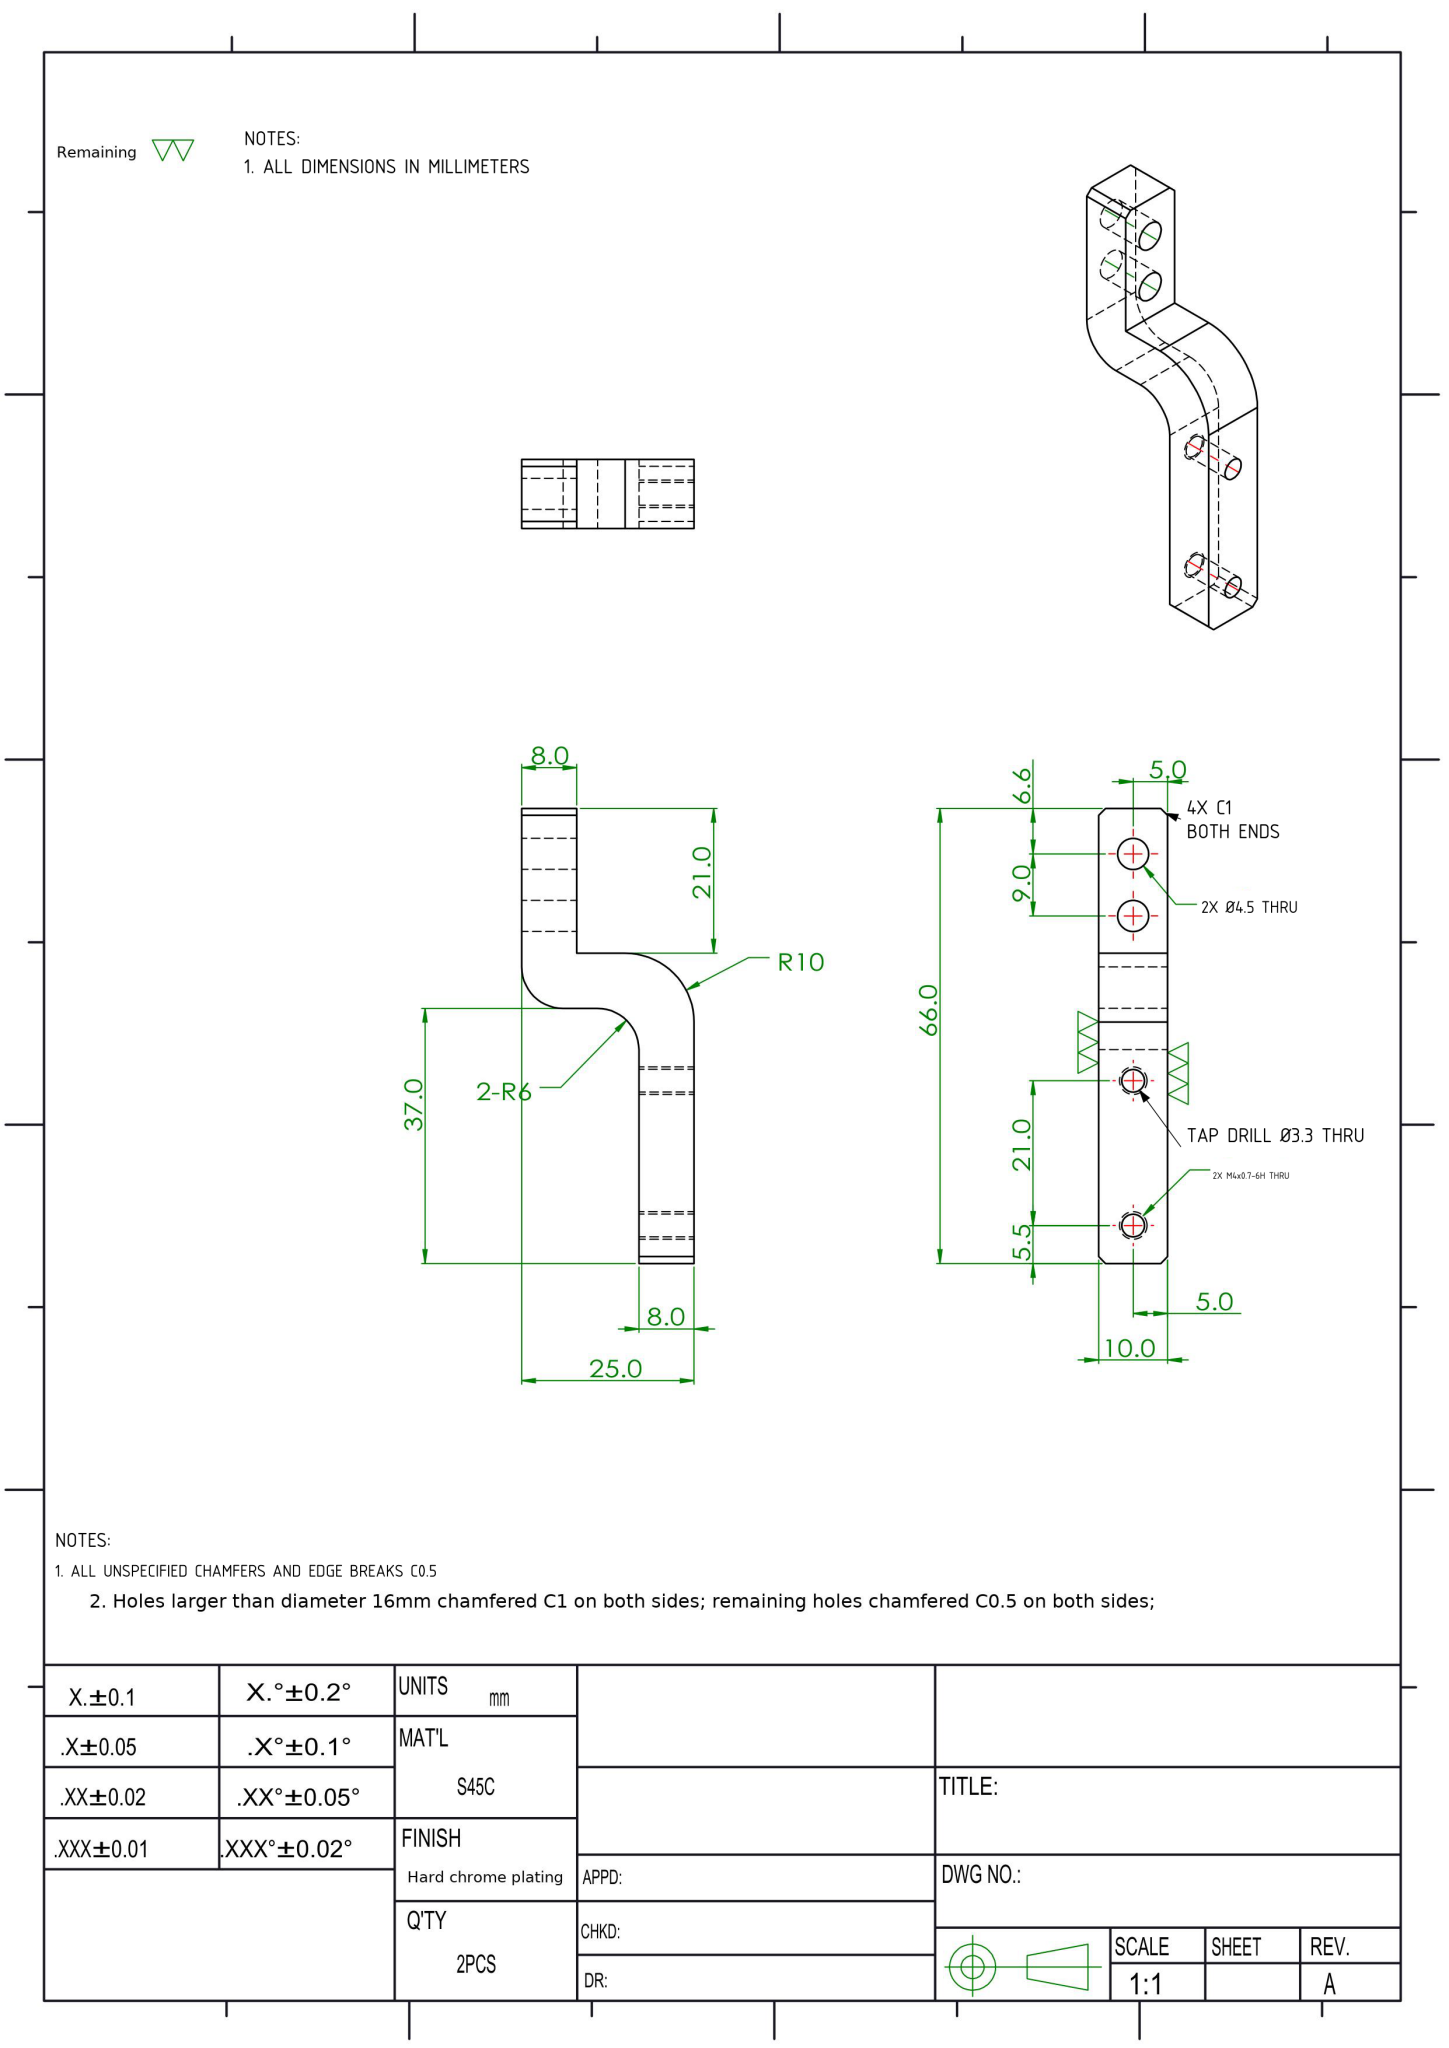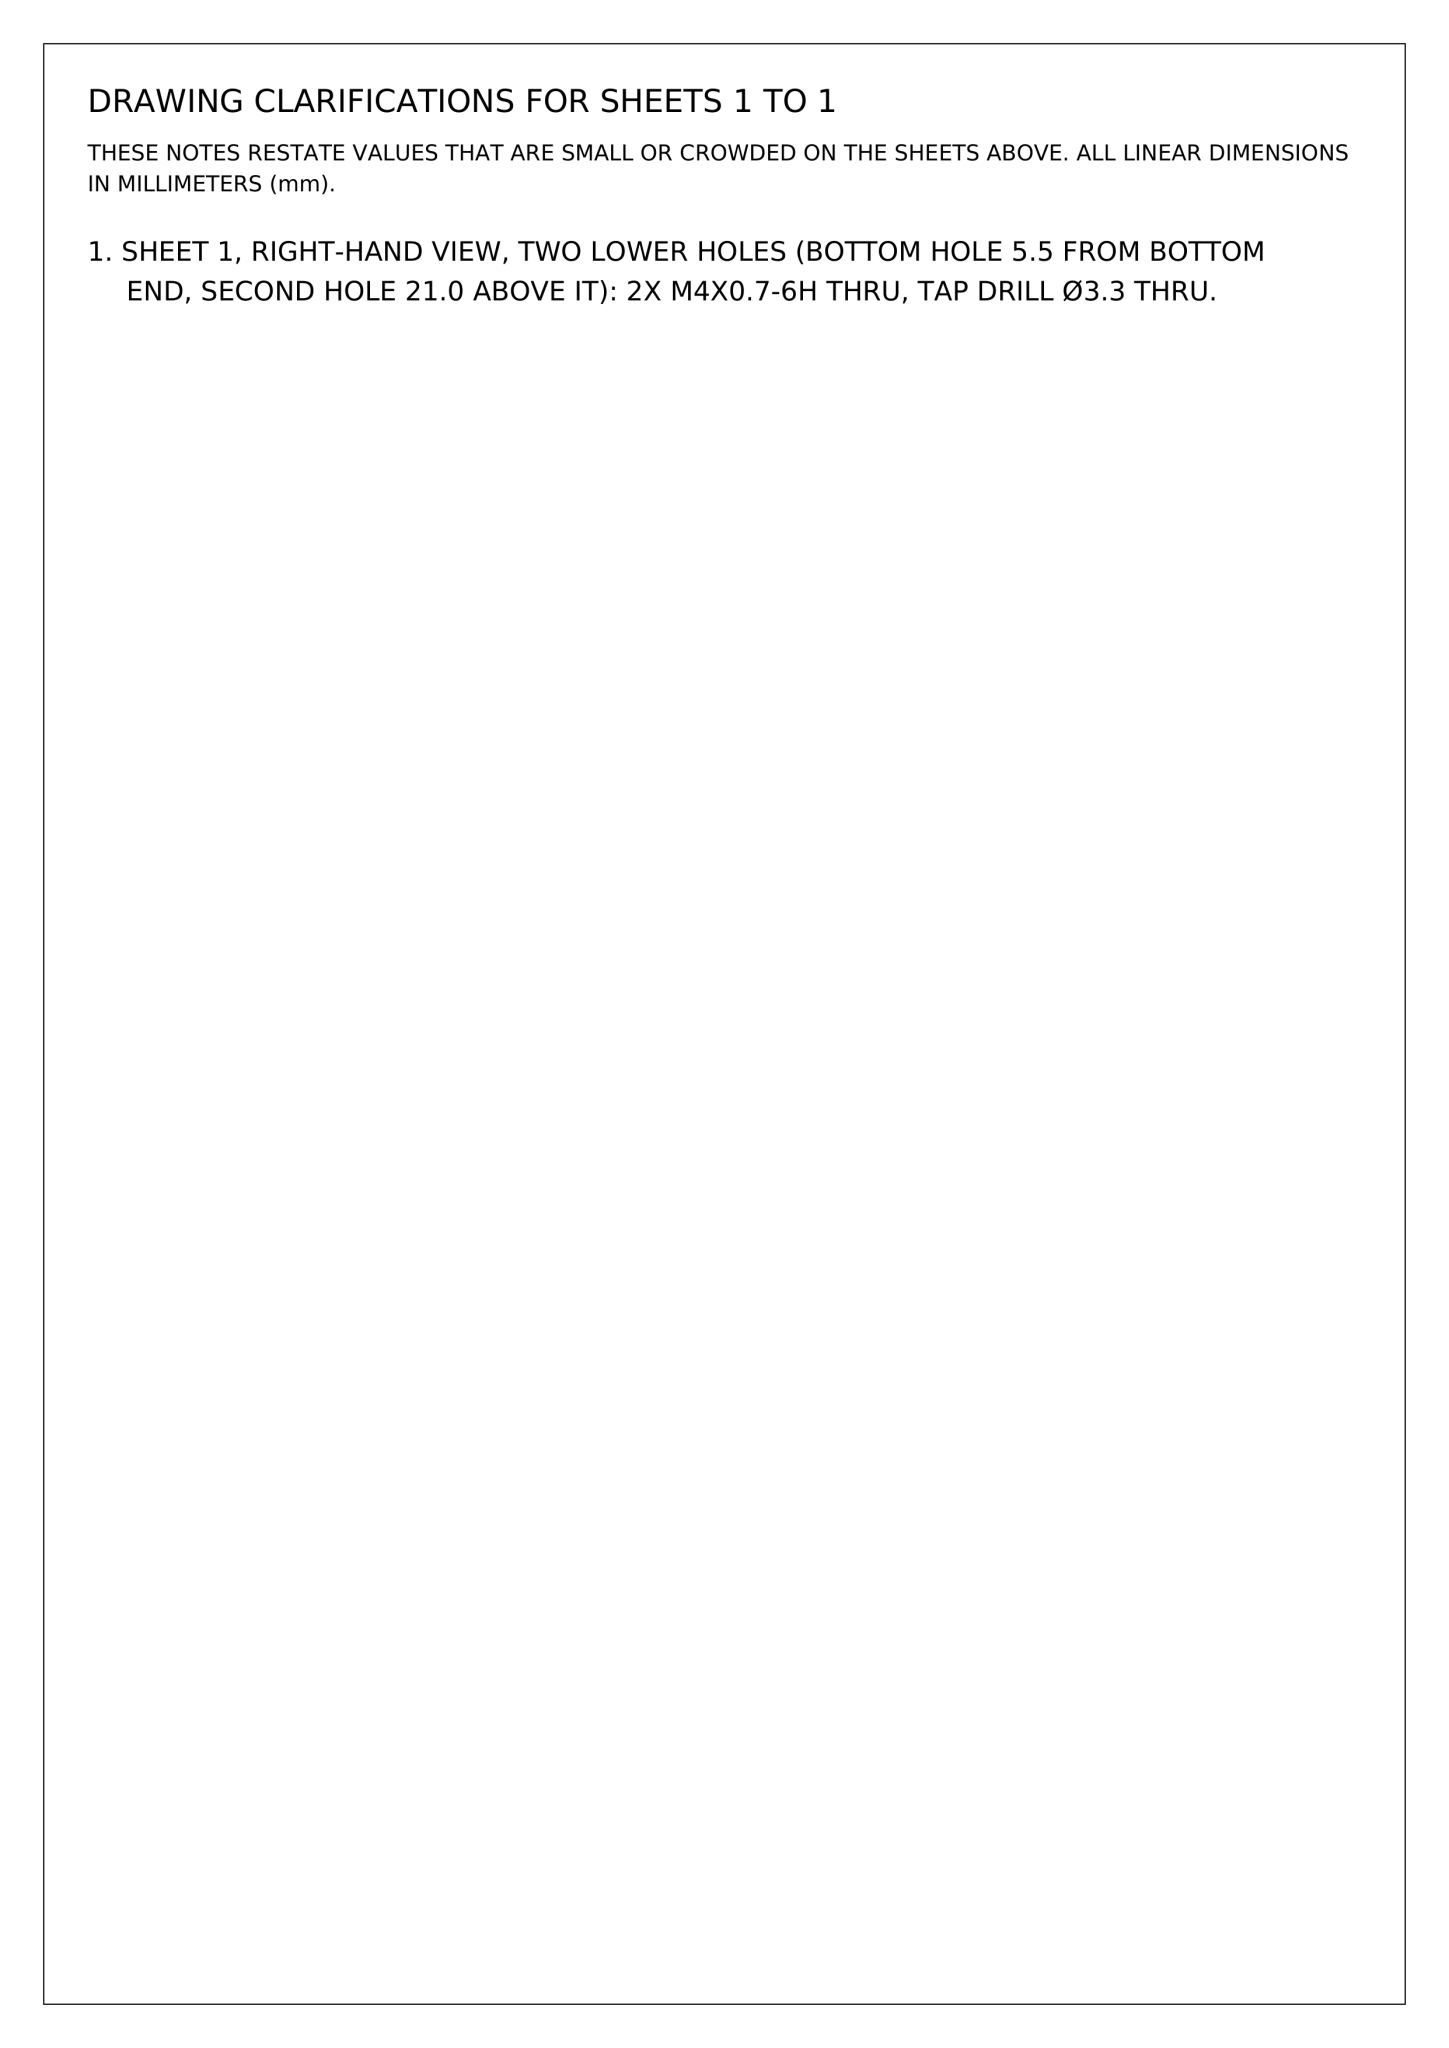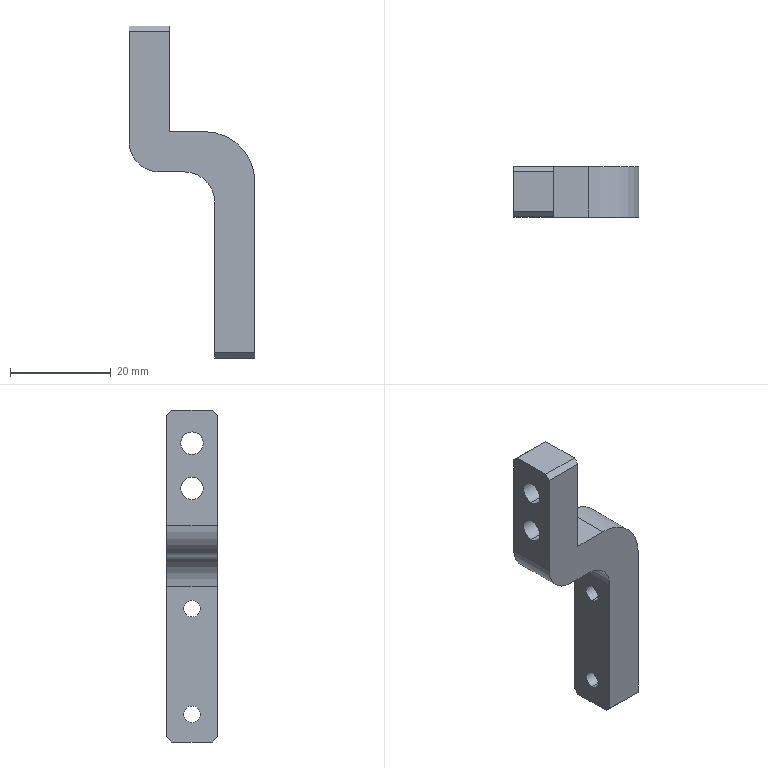Part | NX | mm | S-Curved Four-Hole Mounting Bracket | 1 solid | 25 faces | box 25 x 10 x 66 mm | volume 6018 mm3 | plane 14 | cylinder 11 | commonest cylinder face diameters 3.3 x4 4.5 x4 12 x2 20 x1